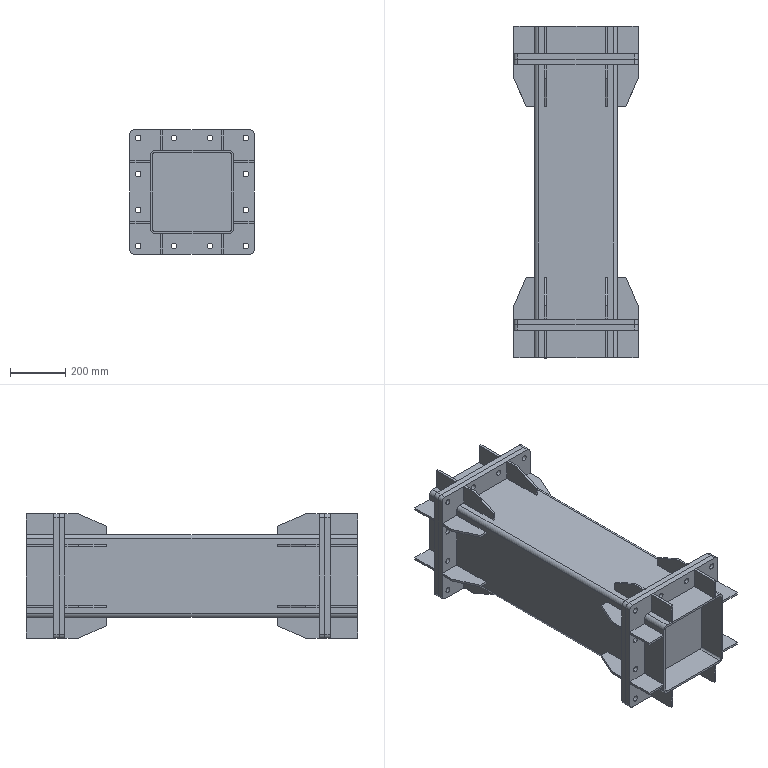Component | SolidWorks | CrossRib-1 | 39 solids | 398 faces | volume 28244731 mm3 | plane 262 | cylinder 136 | commonest cylinder face diameters 21 x96 30 x16 16 x12 32 x12